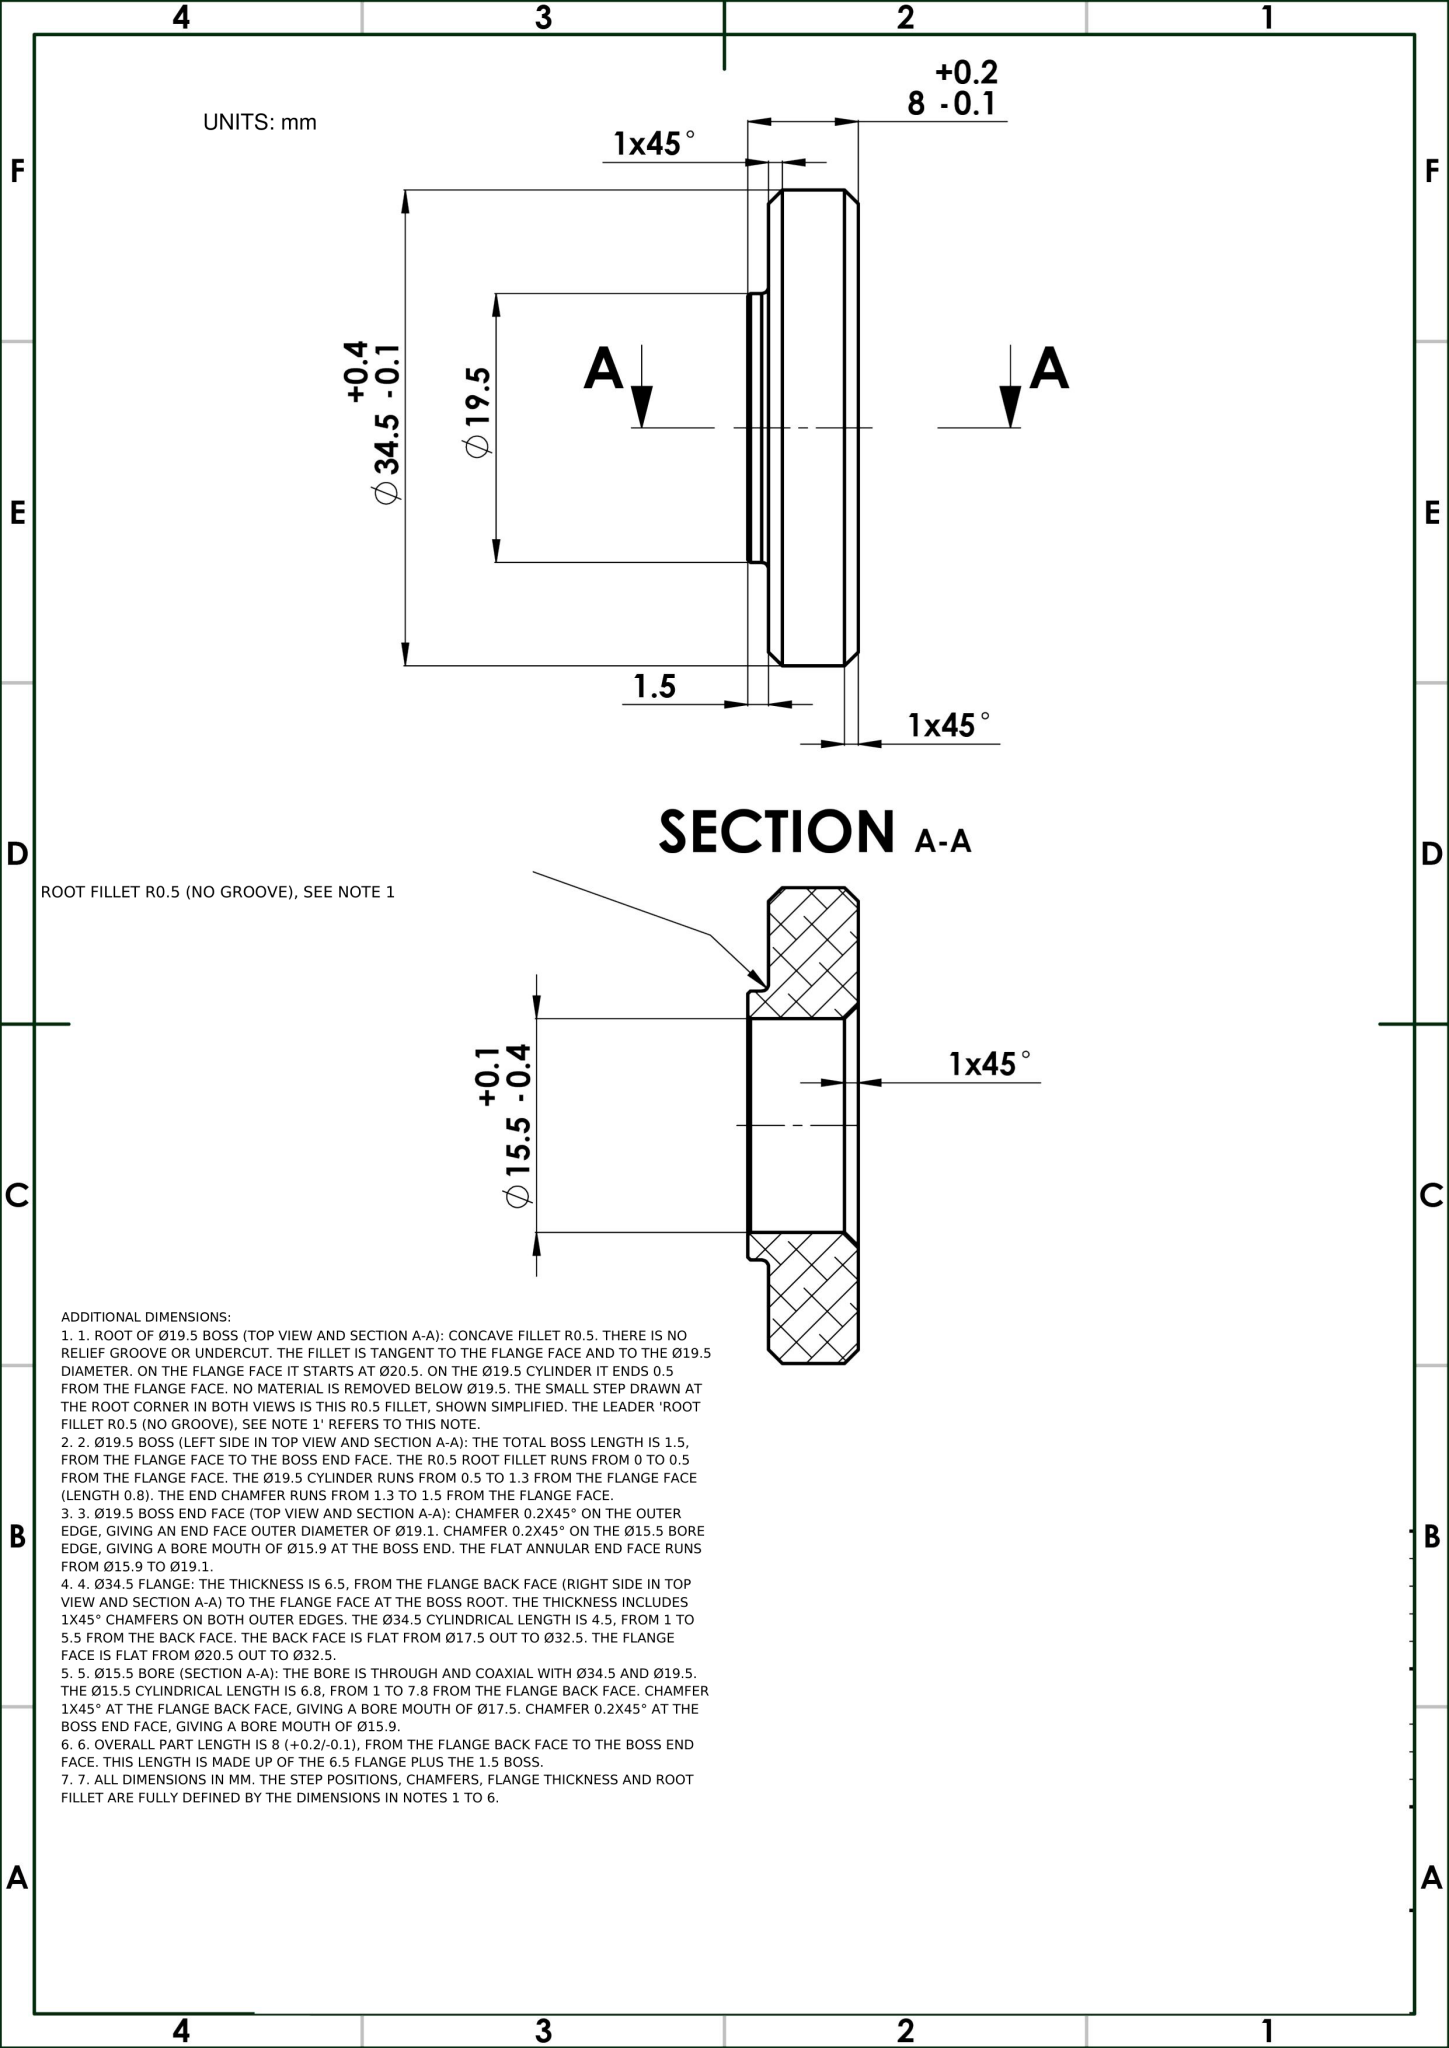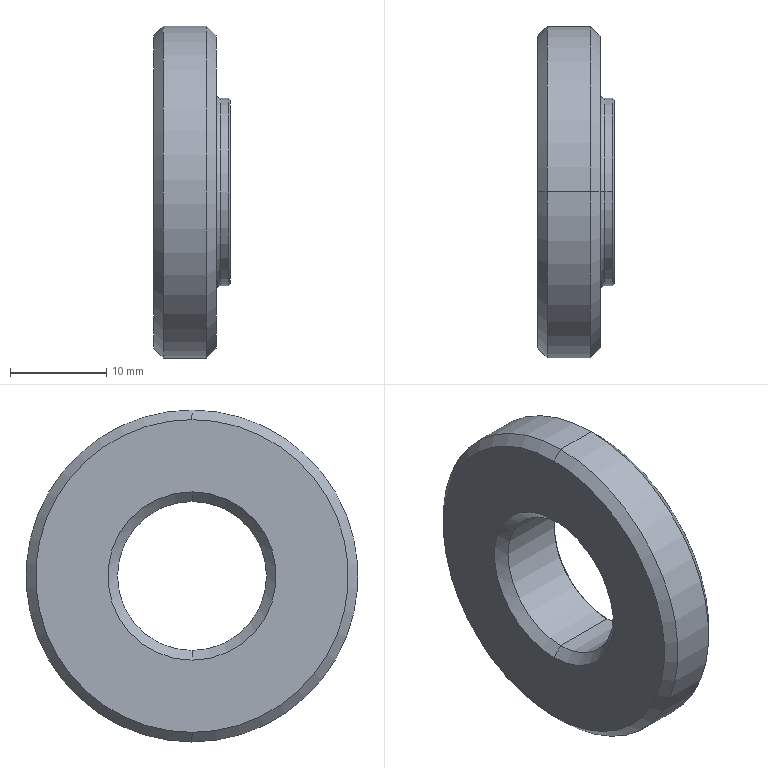Part | NX | mm | 1 solid | 21 faces | box 8 x 34.5 x 34.5 mm | volume 4884 mm3 | cone 10 | cylinder 6 | plane 3 | torus 2 | commonest cylinder face diameters 19.5 x2 15.5 x2 34.5 x2
STEP:
#1=CARTESIAN_POINT('',(7.,0.,9.75));
#2=VERTEX_POINT('',#1);
#3=CARTESIAN_POINT('',(7.,0.,-9.75));
#4=VERTEX_POINT('',#3);
#5=CARTESIAN_POINT('',(7.,0.,0.));
#6=DIRECTION('',(1.,0.,0.));
#7=DIRECTION('',(0.,0.,-1.));
#8=AXIS2_PLACEMENT_3D('',#5,#6,#7);
#9=CIRCLE('',#8,9.75);
#10=EDGE_CURVE('',#2,#4,#9,.T.);
#11=ORIENTED_EDGE('',*,*,#10,.F.);
#12=CARTESIAN_POINT('',(6.5,0.,10.25));
#13=VERTEX_POINT('',#12);
#14=CARTESIAN_POINT('',(7.,0.,10.25));
#15=DIRECTION('',(0.,1.,-0.));
#16=DIRECTION('',(0.,0.,1.));
#17=AXIS2_PLACEMENT_3D('',#14,#15,#16);
#18=CIRCLE('',#17,0.5);
#19=EDGE_CURVE('',#2,#13,#18,.T.);
#20=ORIENTED_EDGE('',*,*,#19,.T.);
#21=CARTESIAN_POINT('',(6.5,0.,-10.25));
#22=VERTEX_POINT('',#21);
#23=CARTESIAN_POINT('',(6.5,0.,0.));
#24=DIRECTION('',(-1.,0.,0.));
#25=DIRECTION('',(0.,0.,-1.));
#26=AXIS2_PLACEMENT_3D('',#23,#24,#25);
#27=CIRCLE('',#26,10.25);
#28=EDGE_CURVE('',#22,#13,#27,.T.);
#29=ORIENTED_EDGE('',*,*,#28,.F.);
#30=CARTESIAN_POINT('',(7.,0.,-10.25));
#31=DIRECTION('',(0.,-1.,0.));
#32=DIRECTION('',(0.,0.,-1.));
#33=AXIS2_PLACEMENT_3D('',#30,#31,#32);
#34=CIRCLE('',#33,0.5);
#35=EDGE_CURVE('',#4,#22,#34,.T.);
#36=ORIENTED_EDGE('',*,*,#35,.F.);
#37=EDGE_LOOP('',(#11,#20,#29,#36));
#38=FACE_OUTER_BOUND('',#37,.T.);
#39=CARTESIAN_POINT('',(7.,0.,0.));
#40=DIRECTION('',(1.,0.,0.));
#41=DIRECTION('',(0.,0.,-1.));
#42=AXIS2_PLACEMENT_3D('',#39,#40,#41);
#43=TOROIDAL_SURFACE('',#42,10.25,0.5);
#44=ADVANCED_FACE('',(#38),#43,.F.);
#45=CARTESIAN_POINT('',(7.8,0.,7.75));
#46=VERTEX_POINT('',#45);
#47=CARTESIAN_POINT('',(7.8,0.,-7.75));
#48=VERTEX_POINT('',#47);
#49=CARTESIAN_POINT('',(7.8,0.,0.));
#50=DIRECTION('',(1.,0.,0.));
#51=DIRECTION('',(0.,0.,1.));
#52=AXIS2_PLACEMENT_3D('',#49,#50,#51);
#53=CIRCLE('',#52,7.75);
#54=EDGE_CURVE('',#46,#48,#53,.T.);
#55=ORIENTED_EDGE('',*,*,#54,.F.);
#56=CARTESIAN_POINT('',(8.,0.,7.95));
#57=VERTEX_POINT('',#56);
#58=CARTESIAN_POINT('',(7.8,0.,7.75));
#59=DIRECTION('',(0.7071,0.,0.7071));
#60=VECTOR('',#59,1000.);
#61=LINE('',#58,#60);
#62=EDGE_CURVE('',#46,#57,#61,.T.);
#63=ORIENTED_EDGE('',*,*,#62,.T.);
#64=CARTESIAN_POINT('',(8.,0.,-7.95));
#65=VERTEX_POINT('',#64);
#66=CARTESIAN_POINT('',(8.,0.,0.));
#67=DIRECTION('',(-1.,0.,0.));
#68=DIRECTION('',(0.,0.,1.));
#69=AXIS2_PLACEMENT_3D('',#66,#67,#68);
#70=CIRCLE('',#69,7.95);
#71=EDGE_CURVE('',#65,#57,#70,.T.);
#72=ORIENTED_EDGE('',*,*,#71,.F.);
#73=CARTESIAN_POINT('',(7.8,0.,-7.75));
#74=DIRECTION('',(0.7071,0.,-0.7071));
#75=VECTOR('',#74,1000.);
#76=LINE('',#73,#75);
#77=EDGE_CURVE('',#48,#65,#76,.T.);
#78=ORIENTED_EDGE('',*,*,#77,.F.);
#79=EDGE_LOOP('',(#55,#63,#72,#78));
#80=FACE_OUTER_BOUND('',#79,.T.);
#81=CARTESIAN_POINT('',(7.8,0.,0.));
#82=DIRECTION('',(1.,0.,0.));
#83=DIRECTION('',(0.,0.,-1.));
#84=AXIS2_PLACEMENT_3D('',#81,#82,#83);
#85=CONICAL_SURFACE('',#84,7.75,0.7854);
#86=ADVANCED_FACE('',(#80),#85,.F.);
#87=CARTESIAN_POINT('',(8.,0.,-9.55));
#88=VERTEX_POINT('',#87);
#89=CARTESIAN_POINT('',(8.,0.,9.55));
#90=VERTEX_POINT('',#89);
#91=CARTESIAN_POINT('',(8.,0.,0.));
#92=DIRECTION('',(1.,0.,0.));
#93=DIRECTION('',(0.,0.,1.));
#94=AXIS2_PLACEMENT_3D('',#91,#92,#93);
#95=CIRCLE('',#94,9.55);
#96=EDGE_CURVE('',#88,#90,#95,.T.);
#97=ORIENTED_EDGE('',*,*,#96,.F.);
#98=CARTESIAN_POINT('',(7.8,0.,-9.75));
#99=VERTEX_POINT('',#98);
#100=CARTESIAN_POINT('',(8.,0.,-9.55));
#101=DIRECTION('',(-0.7071,0.,-0.7071));
#102=VECTOR('',#101,1000.);
#103=LINE('',#100,#102);
#104=EDGE_CURVE('',#88,#99,#103,.T.);
#105=ORIENTED_EDGE('',*,*,#104,.T.);
#106=CARTESIAN_POINT('',(7.8,0.,9.75));
#107=VERTEX_POINT('',#106);
#108=CARTESIAN_POINT('',(7.8,0.,0.));
#109=DIRECTION('',(-1.,0.,0.));
#110=DIRECTION('',(0.,0.,1.));
#111=AXIS2_PLACEMENT_3D('',#108,#109,#110);
#112=CIRCLE('',#111,9.75);
#113=EDGE_CURVE('',#107,#99,#112,.T.);
#114=ORIENTED_EDGE('',*,*,#113,.F.);
#115=CARTESIAN_POINT('',(8.,0.,9.55));
#116=DIRECTION('',(-0.7071,0.,0.7071));
#117=VECTOR('',#116,1000.);
#118=LINE('',#115,#117);
#119=EDGE_CURVE('',#90,#107,#118,.T.);
#120=ORIENTED_EDGE('',*,*,#119,.F.);
#121=EDGE_LOOP('',(#97,#105,#114,#120));
#122=FACE_OUTER_BOUND('',#121,.T.);
#123=CARTESIAN_POINT('',(8.,0.,0.));
#124=DIRECTION('',(-1.,0.,0.));
#125=DIRECTION('',(0.,0.,1.));
#126=AXIS2_PLACEMENT_3D('',#123,#124,#125);
#127=CONICAL_SURFACE('',#126,9.55,0.7854);
#128=ADVANCED_FACE('',(#122),#127,.T.);
#129=CARTESIAN_POINT('',(0.,0.,16.25));
#130=VERTEX_POINT('',#129);
#131=CARTESIAN_POINT('',(0.,0.,-16.25));
#132=VERTEX_POINT('',#131);
#133=CARTESIAN_POINT('',(0.,0.,0.));
#134=DIRECTION('',(-1.,0.,0.));
#135=DIRECTION('',(0.,0.,-1.));
#136=AXIS2_PLACEMENT_3D('',#133,#134,#135);
#137=CIRCLE('',#136,16.25);
#138=EDGE_CURVE('',#130,#132,#137,.T.);
#139=ORIENTED_EDGE('',*,*,#138,.F.);
#140=CARTESIAN_POINT('',(1.,0.,17.25));
#141=VERTEX_POINT('',#140);
#142=CARTESIAN_POINT('',(0.,0.,16.25));
#143=DIRECTION('',(0.7071,0.,0.7071));
#144=VECTOR('',#143,1000.);
#145=LINE('',#142,#144);
#146=EDGE_CURVE('',#130,#141,#145,.T.);
#147=ORIENTED_EDGE('',*,*,#146,.T.);
#148=CARTESIAN_POINT('',(1.,0.,-17.25));
#149=VERTEX_POINT('',#148);
#150=CARTESIAN_POINT('',(1.,0.,0.));
#151=DIRECTION('',(1.,0.,0.));
#152=DIRECTION('',(0.,0.,-1.));
#153=AXIS2_PLACEMENT_3D('',#150,#151,#152);
#154=CIRCLE('',#153,17.25);
#155=EDGE_CURVE('',#149,#141,#154,.T.);
#156=ORIENTED_EDGE('',*,*,#155,.F.);
#157=CARTESIAN_POINT('',(0.,0.,-16.25));
#158=DIRECTION('',(0.7071,0.,-0.7071));
#159=VECTOR('',#158,1000.);
#160=LINE('',#157,#159);
#161=EDGE_CURVE('',#132,#149,#160,.T.);
#162=ORIENTED_EDGE('',*,*,#161,.F.);
#163=EDGE_LOOP('',(#139,#147,#156,#162));
#164=FACE_OUTER_BOUND('',#163,.T.);
#165=CARTESIAN_POINT('',(0.,0.,0.));
#166=DIRECTION('',(1.,0.,0.));
#167=DIRECTION('',(0.,0.,-1.));
#168=AXIS2_PLACEMENT_3D('',#165,#166,#167);
#169=CONICAL_SURFACE('',#168,16.25,0.7854);
#170=ADVANCED_FACE('',(#164),#169,.T.);
#171=CARTESIAN_POINT('',(1.,0.,-7.75));
#172=VERTEX_POINT('',#171);
#173=CARTESIAN_POINT('',(1.,0.,7.75));
#174=VERTEX_POINT('',#173);
#175=CARTESIAN_POINT('',(1.,0.,0.));
#176=DIRECTION('',(-1.,0.,0.));
#177=DIRECTION('',(0.,0.,-1.));
#178=AXIS2_PLACEMENT_3D('',#175,#176,#177);
#179=CIRCLE('',#178,7.75);
#180=EDGE_CURVE('',#172,#174,#179,.T.);
#181=ORIENTED_EDGE('',*,*,#180,.F.);
#182=CARTESIAN_POINT('',(0.,0.,-8.75));
#183=VERTEX_POINT('',#182);
#184=CARTESIAN_POINT('',(0.,0.,-8.75));
#185=DIRECTION('',(-0.7071,0.,-0.7071));
#186=VECTOR('',#185,1000.);
#187=LINE('',#184,#186);
#188=EDGE_CURVE('',#172,#183,#187,.T.);
#189=ORIENTED_EDGE('',*,*,#188,.T.);
#190=CARTESIAN_POINT('',(0.,0.,8.75));
#191=VERTEX_POINT('',#190);
#192=CARTESIAN_POINT('',(0.,0.,0.));
#193=DIRECTION('',(1.,0.,0.));
#194=DIRECTION('',(0.,0.,-1.));
#195=AXIS2_PLACEMENT_3D('',#192,#193,#194);
#196=CIRCLE('',#195,8.75);
#197=EDGE_CURVE('',#191,#183,#196,.T.);
#198=ORIENTED_EDGE('',*,*,#197,.F.);
#199=CARTESIAN_POINT('',(0.,0.,8.75));
#200=DIRECTION('',(-0.7071,0.,0.7071));
#201=VECTOR('',#200,1000.);
#202=LINE('',#199,#201);
#203=EDGE_CURVE('',#174,#191,#202,.T.);
#204=ORIENTED_EDGE('',*,*,#203,.F.);
#205=EDGE_LOOP('',(#181,#189,#198,#204));
#206=FACE_OUTER_BOUND('',#205,.T.);
#207=CARTESIAN_POINT('',(0.,0.,0.));
#208=DIRECTION('',(-1.,0.,0.));
#209=DIRECTION('',(0.,0.,1.));
#210=AXIS2_PLACEMENT_3D('',#207,#208,#209);
#211=CONICAL_SURFACE('',#210,8.75,0.7854);
#212=ADVANCED_FACE('',(#206),#211,.F.);
#213=CARTESIAN_POINT('',(6.5,0.,-16.25));
#214=VERTEX_POINT('',#213);
#215=CARTESIAN_POINT('',(6.5,0.,16.25));
#216=VERTEX_POINT('',#215);
#217=CARTESIAN_POINT('',(6.5,0.,0.));
#218=DIRECTION('',(1.,0.,0.));
#219=DIRECTION('',(0.,0.,-1.));
#220=AXIS2_PLACEMENT_3D('',#217,#218,#219);
#221=CIRCLE('',#220,16.25);
#222=EDGE_CURVE('',#214,#216,#221,.T.);
#223=ORIENTED_EDGE('',*,*,#222,.F.);
#224=CARTESIAN_POINT('',(5.5,0.,-17.25));
#225=VERTEX_POINT('',#224);
#226=CARTESIAN_POINT('',(6.5,0.,-16.25));
#227=DIRECTION('',(-0.7071,0.,-0.7071));
#228=VECTOR('',#227,1000.);
#229=LINE('',#226,#228);
#230=EDGE_CURVE('',#214,#225,#229,.T.);
#231=ORIENTED_EDGE('',*,*,#230,.T.);
#232=CARTESIAN_POINT('',(5.5,0.,17.25));
#233=VERTEX_POINT('',#232);
#234=CARTESIAN_POINT('',(5.5,0.,0.));
#235=DIRECTION('',(-1.,0.,0.));
#236=DIRECTION('',(0.,0.,-1.));
#237=AXIS2_PLACEMENT_3D('',#234,#235,#236);
#238=CIRCLE('',#237,17.25);
#239=EDGE_CURVE('',#233,#225,#238,.T.);
#240=ORIENTED_EDGE('',*,*,#239,.F.);
#241=CARTESIAN_POINT('',(6.5,0.,16.25));
#242=DIRECTION('',(-0.7071,0.,0.7071));
#243=VECTOR('',#242,1000.);
#244=LINE('',#241,#243);
#245=EDGE_CURVE('',#216,#233,#244,.T.);
#246=ORIENTED_EDGE('',*,*,#245,.F.);
#247=EDGE_LOOP('',(#223,#231,#240,#246));
#248=FACE_OUTER_BOUND('',#247,.T.);
#249=CARTESIAN_POINT('',(6.5,0.,0.));
#250=DIRECTION('',(-1.,0.,0.));
#251=DIRECTION('',(0.,0.,1.));
#252=AXIS2_PLACEMENT_3D('',#249,#250,#251);
#253=CONICAL_SURFACE('',#252,16.25,0.7854);
#254=ADVANCED_FACE('',(#248),#253,.T.);
#255=CARTESIAN_POINT('',(7.,0.,0.));
#256=DIRECTION('',(1.,0.,0.));
#257=DIRECTION('',(0.,0.,-1.));
#258=AXIS2_PLACEMENT_3D('',#255,#256,#257);
#259=CIRCLE('',#258,9.75);
#260=EDGE_CURVE('',#4,#2,#259,.T.);
#261=ORIENTED_EDGE('',*,*,#260,.T.);
#262=CARTESIAN_POINT('',(6.5,0.,9.75));
#263=DIRECTION('',(1.,0.,0.));
#264=VECTOR('',#263,1000.);
#265=LINE('',#262,#264);
#266=EDGE_CURVE('',#2,#107,#265,.T.);
#267=ORIENTED_EDGE('',*,*,#266,.T.);
#268=ORIENTED_EDGE('',*,*,#113,.T.);
#269=CARTESIAN_POINT('',(6.5,0.,-9.75));
#270=DIRECTION('',(1.,0.,0.));
#271=VECTOR('',#270,1000.);
#272=LINE('',#269,#271);
#273=EDGE_CURVE('',#4,#99,#272,.T.);
#274=ORIENTED_EDGE('',*,*,#273,.F.);
#275=EDGE_LOOP('',(#261,#267,#268,#274));
#276=FACE_OUTER_BOUND('',#275,.T.);
#277=CARTESIAN_POINT('',(6.5,0.,0.));
#278=DIRECTION('',(1.,0.,0.));
#279=DIRECTION('',(0.,0.,-1.));
#280=AXIS2_PLACEMENT_3D('',#277,#278,#279);
#281=CYLINDRICAL_SURFACE('',#280,9.75);
#282=ADVANCED_FACE('',(#276),#281,.T.);
#283=ORIENTED_EDGE('',*,*,#180,.T.);
#284=CARTESIAN_POINT('',(-2.,0.,7.75));
#285=DIRECTION('',(1.,0.,0.));
#286=VECTOR('',#285,1000.);
#287=LINE('',#284,#286);
#288=EDGE_CURVE('',#174,#46,#287,.T.);
#289=ORIENTED_EDGE('',*,*,#288,.T.);
#290=ORIENTED_EDGE('',*,*,#54,.T.);
#291=CARTESIAN_POINT('',(-2.,0.,-7.75));
#292=DIRECTION('',(1.,0.,0.));
#293=VECTOR('',#292,1000.);
#294=LINE('',#291,#293);
#295=EDGE_CURVE('',#172,#48,#294,.T.);
#296=ORIENTED_EDGE('',*,*,#295,.F.);
#297=EDGE_LOOP('',(#283,#289,#290,#296));
#298=FACE_OUTER_BOUND('',#297,.T.);
#299=CARTESIAN_POINT('',(-2.,0.,0.));
#300=DIRECTION('',(1.,0.,0.));
#301=DIRECTION('',(0.,0.,-1.));
#302=AXIS2_PLACEMENT_3D('',#299,#300,#301);
#303=CYLINDRICAL_SURFACE('',#302,7.75);
#304=ADVANCED_FACE('',(#298),#303,.F.);
#305=ORIENTED_EDGE('',*,*,#239,.T.);
#306=CARTESIAN_POINT('',(0.,0.,-17.25));
#307=DIRECTION('',(-1.,0.,0.));
#308=VECTOR('',#307,1000.);
#309=LINE('',#306,#308);
#310=EDGE_CURVE('',#225,#149,#309,.T.);
#311=ORIENTED_EDGE('',*,*,#310,.T.);
#312=ORIENTED_EDGE('',*,*,#155,.T.);
#313=CARTESIAN_POINT('',(0.,0.,17.25));
#314=DIRECTION('',(-1.,0.,0.));
#315=VECTOR('',#314,1000.);
#316=LINE('',#313,#315);
#317=EDGE_CURVE('',#233,#141,#316,.T.);
#318=ORIENTED_EDGE('',*,*,#317,.F.);
#319=EDGE_LOOP('',(#305,#311,#312,#318));
#320=FACE_OUTER_BOUND('',#319,.T.);
#321=CARTESIAN_POINT('',(0.,0.,0.));
#322=DIRECTION('',(-1.,0.,0.));
#323=DIRECTION('',(0.,0.,1.));
#324=AXIS2_PLACEMENT_3D('',#321,#322,#323);
#325=CYLINDRICAL_SURFACE('',#324,17.25);
#326=ADVANCED_FACE('',(#320),#325,.T.);
#327=ORIENTED_EDGE('',*,*,#310,.F.);
#328=CARTESIAN_POINT('',(5.5,0.,0.));
#329=DIRECTION('',(-1.,0.,0.));
#330=DIRECTION('',(0.,0.,-1.));
#331=AXIS2_PLACEMENT_3D('',#328,#329,#330);
#332=CIRCLE('',#331,17.25);
#333=EDGE_CURVE('',#225,#233,#332,.T.);
#334=ORIENTED_EDGE('',*,*,#333,.T.);
#335=ORIENTED_EDGE('',*,*,#317,.T.);
#336=CARTESIAN_POINT('',(1.,0.,0.));
#337=DIRECTION('',(1.,0.,0.));
#338=DIRECTION('',(0.,0.,-1.));
#339=AXIS2_PLACEMENT_3D('',#336,#337,#338);
#340=CIRCLE('',#339,17.25);
#341=EDGE_CURVE('',#141,#149,#340,.T.);
#342=ORIENTED_EDGE('',*,*,#341,.T.);
#343=EDGE_LOOP('',(#327,#334,#335,#342));
#344=FACE_OUTER_BOUND('',#343,.T.);
#345=CARTESIAN_POINT('',(0.,0.,0.));
#346=DIRECTION('',(-1.,0.,0.));
#347=DIRECTION('',(0.,0.,1.));
#348=AXIS2_PLACEMENT_3D('',#345,#346,#347);
#349=CYLINDRICAL_SURFACE('',#348,17.25);
#350=ADVANCED_FACE('',(#344),#349,.T.);
#351=CARTESIAN_POINT('',(8.,0.,0.));
#352=DIRECTION('',(1.,0.,0.));
#353=DIRECTION('',(0.,0.,1.));
#354=AXIS2_PLACEMENT_3D('',#351,#352,#353);
#355=CIRCLE('',#354,9.55);
#356=EDGE_CURVE('',#90,#88,#355,.T.);
#357=ORIENTED_EDGE('',*,*,#356,.T.);
#358=ORIENTED_EDGE('',*,*,#96,.T.);
#359=EDGE_LOOP('',(#357,#358));
#360=FACE_OUTER_BOUND('',#359,.T.);
#361=ORIENTED_EDGE('',*,*,#71,.T.);
#362=CARTESIAN_POINT('',(8.,0.,0.));
#363=DIRECTION('',(-1.,0.,0.));
#364=DIRECTION('',(0.,0.,1.));
#365=AXIS2_PLACEMENT_3D('',#362,#363,#364);
#366=CIRCLE('',#365,7.95);
#367=EDGE_CURVE('',#57,#65,#366,.T.);
#368=ORIENTED_EDGE('',*,*,#367,.T.);
#369=EDGE_LOOP('',(#361,#368));
#370=FACE_BOUND('',#369,.T.);
#371=CARTESIAN_POINT('',(8.,0.,0.));
#372=DIRECTION('',(-1.,0.,0.));
#373=DIRECTION('',(0.,0.,1.));
#374=AXIS2_PLACEMENT_3D('',#371,#372,#373);
#375=PLANE('',#374);
#376=ADVANCED_FACE('',(#360,#370),#375,.F.);
#377=ORIENTED_EDGE('',*,*,#197,.T.);
#378=CARTESIAN_POINT('',(0.,0.,0.));
#379=DIRECTION('',(1.,0.,0.));
#380=DIRECTION('',(0.,0.,-1.));
#381=AXIS2_PLACEMENT_3D('',#378,#379,#380);
#382=CIRCLE('',#381,8.75);
#383=EDGE_CURVE('',#183,#191,#382,.T.);
#384=ORIENTED_EDGE('',*,*,#383,.T.);
#385=EDGE_LOOP('',(#377,#384));
#386=FACE_BOUND('',#385,.T.);
#387=CARTESIAN_POINT('',(0.,0.,0.));
#388=DIRECTION('',(-1.,0.,0.));
#389=DIRECTION('',(0.,0.,-1.));
#390=AXIS2_PLACEMENT_3D('',#387,#388,#389);
#391=CIRCLE('',#390,16.25);
#392=EDGE_CURVE('',#132,#130,#391,.T.);
#393=ORIENTED_EDGE('',*,*,#392,.T.);
#394=ORIENTED_EDGE('',*,*,#138,.T.);
#395=EDGE_LOOP('',(#393,#394));
#396=FACE_OUTER_BOUND('',#395,.T.);
#397=CARTESIAN_POINT('',(0.,0.,0.));
#398=DIRECTION('',(1.,0.,0.));
#399=DIRECTION('',(0.,0.,-1.));
#400=AXIS2_PLACEMENT_3D('',#397,#398,#399);
#401=PLANE('',#400);
#402=ADVANCED_FACE('',(#386,#396),#401,.F.);
#403=ORIENTED_EDGE('',*,*,#288,.F.);
#404=CARTESIAN_POINT('',(1.,0.,0.));
#405=DIRECTION('',(-1.,0.,0.));
#406=DIRECTION('',(0.,0.,-1.));
#407=AXIS2_PLACEMENT_3D('',#404,#405,#406);
#408=CIRCLE('',#407,7.75);
#409=EDGE_CURVE('',#174,#172,#408,.T.);
#410=ORIENTED_EDGE('',*,*,#409,.T.);
#411=ORIENTED_EDGE('',*,*,#295,.T.);
#412=CARTESIAN_POINT('',(7.8,0.,0.));
#413=DIRECTION('',(1.,0.,0.));
#414=DIRECTION('',(0.,0.,1.));
#415=AXIS2_PLACEMENT_3D('',#412,#413,#414);
#416=CIRCLE('',#415,7.75);
#417=EDGE_CURVE('',#48,#46,#416,.T.);
#418=ORIENTED_EDGE('',*,*,#417,.T.);
#419=EDGE_LOOP('',(#403,#410,#411,#418));
#420=FACE_OUTER_BOUND('',#419,.T.);
#421=CARTESIAN_POINT('',(-2.,0.,0.));
#422=DIRECTION('',(1.,0.,0.));
#423=DIRECTION('',(0.,0.,-1.));
#424=AXIS2_PLACEMENT_3D('',#421,#422,#423);
#425=CYLINDRICAL_SURFACE('',#424,7.75);
#426=ADVANCED_FACE('',(#420),#425,.F.);
#427=ORIENTED_EDGE('',*,*,#266,.F.);
#428=ORIENTED_EDGE('',*,*,#10,.T.);
#429=ORIENTED_EDGE('',*,*,#273,.T.);
#430=CARTESIAN_POINT('',(7.8,0.,0.));
#431=DIRECTION('',(-1.,0.,0.));
#432=DIRECTION('',(0.,0.,1.));
#433=AXIS2_PLACEMENT_3D('',#430,#431,#432);
#434=CIRCLE('',#433,9.75);
#435=EDGE_CURVE('',#99,#107,#434,.T.);
#436=ORIENTED_EDGE('',*,*,#435,.T.);
#437=EDGE_LOOP('',(#427,#428,#429,#436));
#438=FACE_OUTER_BOUND('',#437,.T.);
#439=CARTESIAN_POINT('',(6.5,0.,0.));
#440=DIRECTION('',(1.,0.,0.));
#441=DIRECTION('',(0.,0.,-1.));
#442=AXIS2_PLACEMENT_3D('',#439,#440,#441);
#443=CYLINDRICAL_SURFACE('',#442,9.75);
#444=ADVANCED_FACE('',(#438),#443,.T.);
#445=ORIENTED_EDGE('',*,*,#28,.T.);
#446=CARTESIAN_POINT('',(6.5,0.,0.));
#447=DIRECTION('',(-1.,0.,0.));
#448=DIRECTION('',(0.,0.,-1.));
#449=AXIS2_PLACEMENT_3D('',#446,#447,#448);
#450=CIRCLE('',#449,10.25);
#451=EDGE_CURVE('',#13,#22,#450,.T.);
#452=ORIENTED_EDGE('',*,*,#451,.T.);
#453=EDGE_LOOP('',(#445,#452));
#454=FACE_BOUND('',#453,.T.);
#455=CARTESIAN_POINT('',(6.5,0.,0.));
#456=DIRECTION('',(1.,0.,0.));
#457=DIRECTION('',(0.,0.,-1.));
#458=AXIS2_PLACEMENT_3D('',#455,#456,#457);
#459=CIRCLE('',#458,16.25);
#460=EDGE_CURVE('',#216,#214,#459,.T.);
#461=ORIENTED_EDGE('',*,*,#460,.T.);
#462=ORIENTED_EDGE('',*,*,#222,.T.);
#463=EDGE_LOOP('',(#461,#462));
#464=FACE_OUTER_BOUND('',#463,.T.);
#465=CARTESIAN_POINT('',(6.5,0.,0.));
#466=DIRECTION('',(1.,0.,0.));
#467=DIRECTION('',(0.,0.,-1.));
#468=AXIS2_PLACEMENT_3D('',#465,#466,#467);
#469=PLANE('',#468);
#470=ADVANCED_FACE('',(#454,#464),#469,.T.);
#471=ORIENTED_EDGE('',*,*,#230,.F.);
#472=ORIENTED_EDGE('',*,*,#460,.F.);
#473=ORIENTED_EDGE('',*,*,#245,.T.);
#474=ORIENTED_EDGE('',*,*,#333,.F.);
#475=EDGE_LOOP('',(#471,#472,#473,#474));
#476=FACE_OUTER_BOUND('',#475,.T.);
#477=CARTESIAN_POINT('',(6.5,0.,0.));
#478=DIRECTION('',(-1.,0.,0.));
#479=DIRECTION('',(0.,0.,1.));
#480=AXIS2_PLACEMENT_3D('',#477,#478,#479);
#481=CONICAL_SURFACE('',#480,16.25,0.7854);
#482=ADVANCED_FACE('',(#476),#481,.T.);
#483=ORIENTED_EDGE('',*,*,#188,.F.);
#484=ORIENTED_EDGE('',*,*,#409,.F.);
#485=ORIENTED_EDGE('',*,*,#203,.T.);
#486=ORIENTED_EDGE('',*,*,#383,.F.);
#487=EDGE_LOOP('',(#483,#484,#485,#486));
#488=FACE_OUTER_BOUND('',#487,.T.);
#489=CARTESIAN_POINT('',(0.,0.,0.));
#490=DIRECTION('',(-1.,0.,0.));
#491=DIRECTION('',(0.,0.,1.));
#492=AXIS2_PLACEMENT_3D('',#489,#490,#491);
#493=CONICAL_SURFACE('',#492,8.75,0.7854);
#494=ADVANCED_FACE('',(#488),#493,.F.);
#495=ORIENTED_EDGE('',*,*,#146,.F.);
#496=ORIENTED_EDGE('',*,*,#392,.F.);
#497=ORIENTED_EDGE('',*,*,#161,.T.);
#498=ORIENTED_EDGE('',*,*,#341,.F.);
#499=EDGE_LOOP('',(#495,#496,#497,#498));
#500=FACE_OUTER_BOUND('',#499,.T.);
#501=CARTESIAN_POINT('',(0.,0.,0.));
#502=DIRECTION('',(1.,0.,0.));
#503=DIRECTION('',(0.,0.,-1.));
#504=AXIS2_PLACEMENT_3D('',#501,#502,#503);
#505=CONICAL_SURFACE('',#504,16.25,0.7854);
#506=ADVANCED_FACE('',(#500),#505,.T.);
#507=ORIENTED_EDGE('',*,*,#104,.F.);
#508=ORIENTED_EDGE('',*,*,#356,.F.);
#509=ORIENTED_EDGE('',*,*,#119,.T.);
#510=ORIENTED_EDGE('',*,*,#435,.F.);
#511=EDGE_LOOP('',(#507,#508,#509,#510));
#512=FACE_OUTER_BOUND('',#511,.T.);
#513=CARTESIAN_POINT('',(8.,0.,0.));
#514=DIRECTION('',(-1.,0.,0.));
#515=DIRECTION('',(0.,0.,1.));
#516=AXIS2_PLACEMENT_3D('',#513,#514,#515);
#517=CONICAL_SURFACE('',#516,9.55,0.7854);
#518=ADVANCED_FACE('',(#512),#517,.T.);
#519=ORIENTED_EDGE('',*,*,#62,.F.);
#520=ORIENTED_EDGE('',*,*,#417,.F.);
#521=ORIENTED_EDGE('',*,*,#77,.T.);
#522=ORIENTED_EDGE('',*,*,#367,.F.);
#523=EDGE_LOOP('',(#519,#520,#521,#522));
#524=FACE_OUTER_BOUND('',#523,.T.);
#525=CARTESIAN_POINT('',(7.8,0.,0.));
#526=DIRECTION('',(1.,0.,0.));
#527=DIRECTION('',(0.,0.,-1.));
#528=AXIS2_PLACEMENT_3D('',#525,#526,#527);
#529=CONICAL_SURFACE('',#528,7.75,0.7854);
#530=ADVANCED_FACE('',(#524),#529,.F.);
#531=ORIENTED_EDGE('',*,*,#19,.F.);
#532=ORIENTED_EDGE('',*,*,#260,.F.);
#533=ORIENTED_EDGE('',*,*,#35,.T.);
#534=ORIENTED_EDGE('',*,*,#451,.F.);
#535=EDGE_LOOP('',(#531,#532,#533,#534));
#536=FACE_OUTER_BOUND('',#535,.T.);
#537=CARTESIAN_POINT('',(7.,0.,0.));
#538=DIRECTION('',(1.,0.,0.));
#539=DIRECTION('',(0.,0.,-1.));
#540=AXIS2_PLACEMENT_3D('',#537,#538,#539);
#541=TOROIDAL_SURFACE('',#540,10.25,0.5);
#542=ADVANCED_FACE('',(#536),#541,.F.);
#543=CLOSED_SHELL('',(#44,#86,#128,#170,#212,#254,#282,#304,#326,#350,#376,#402,#426,#444,#470,#482,#494,#506,#518,#530,#542));
#544=MANIFOLD_SOLID_BREP('',#543);
#545=CARTESIAN_POINT('',(0.,0.,0.));
#546=DIRECTION('',(0.,0.,1.));
#547=DIRECTION('',(1.,0.,0.));
#548=AXIS2_PLACEMENT_3D('',#545,#546,#547);
#549=(LENGTH_UNIT()NAMED_UNIT(*)SI_UNIT(.MILLI.,.METRE.));
#550=UNCERTAINTY_MEASURE_WITH_UNIT(LENGTH_MEASURE(0.00001),#549,'','');
#551=(NAMED_UNIT(*)PLANE_ANGLE_UNIT()SI_UNIT($,.RADIAN.));
#552=(NAMED_UNIT(*)SI_UNIT($,.STERADIAN.)SOLID_ANGLE_UNIT());
#553=(GEOMETRIC_REPRESENTATION_CONTEXT(3)GLOBAL_UNCERTAINTY_ASSIGNED_CONTEXT((#550))GLOBAL_UNIT_ASSIGNED_CONTEXT((#549,#551,#552))REPRESENTATION_CONTEXT('',''));
#554=ADVANCED_BREP_SHAPE_REPRESENTATION('',(#544,#548),#553);